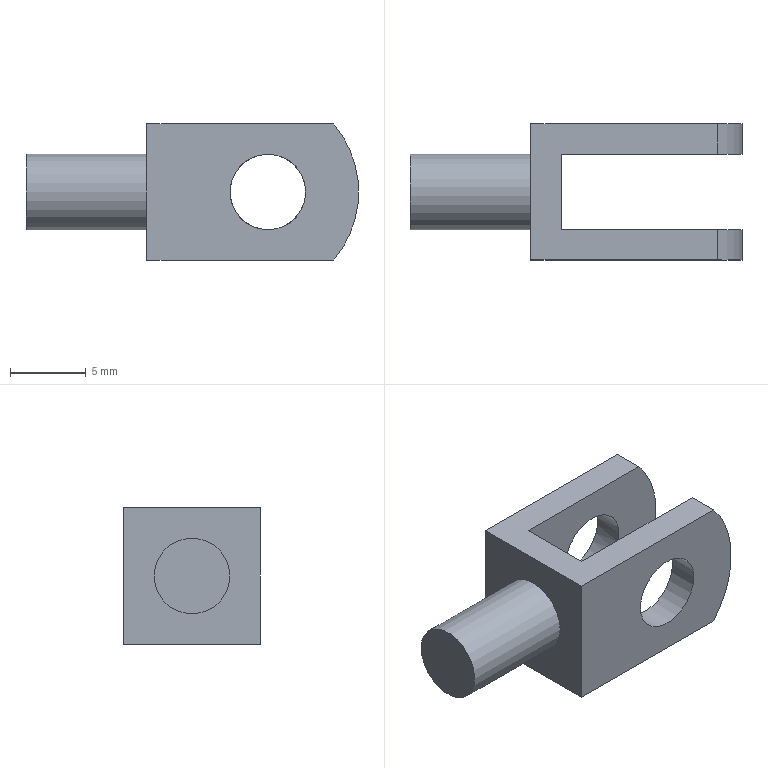Component | NX | PISTON_STRAIGHT_ROD_CONNECTING_BLOCK | 1 solid | 18 faces | volume 654 mm3 | plane 11 | cylinder 7 | commonest cylinder face diameters 14 x4 5 x3